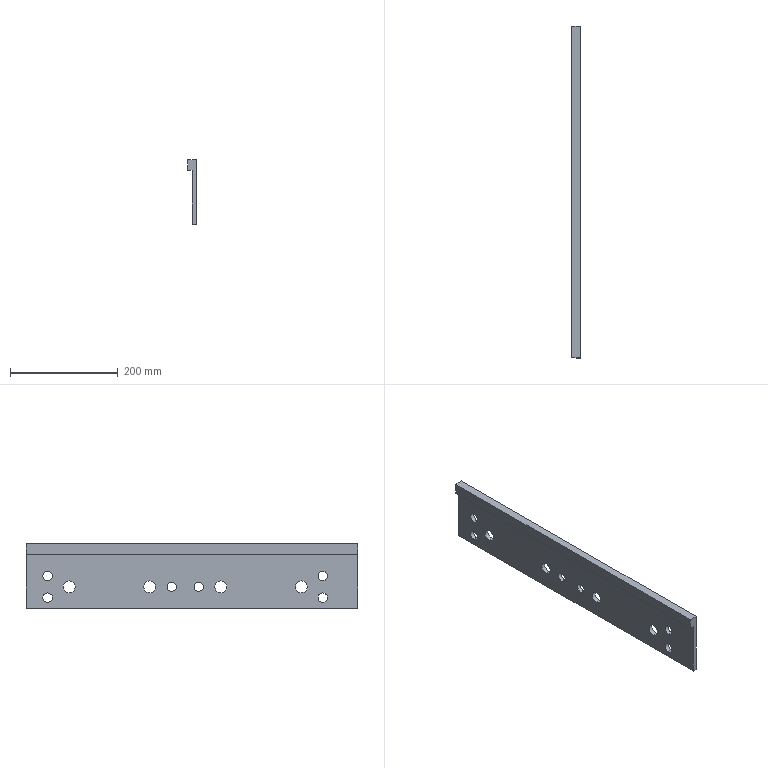Component | SolidWorks | JF21-80.1-1-3(_)-1-SOLID67-1 | 1 solid | 28 faces | box 15 x 615 x 120 mm | volume 623522 mm3 | cylinder 20 | plane 8 | commonest cylinder face diameters 17.5 x12 22 x8
STEP:
#1=COLOUR_RGB('',0.7922,0.8196,0.9333);
#2=FILL_AREA_STYLE_COLOUR('',#1);
#3=FILL_AREA_STYLE('',(#2));
#4=SURFACE_STYLE_FILL_AREA(#3);
#5=SURFACE_SIDE_STYLE('',(#4));
#6=SURFACE_STYLE_USAGE(.BOTH.,#5);
#7=PRESENTATION_STYLE_ASSIGNMENT((#6));
#8=CARTESIAN_POINT('',(15.453,-16.339,5.236));
#9=VERTEX_POINT('',#8);
#10=CARTESIAN_POINT('',(15.453,-16.339,4.37));
#11=VERTEX_POINT('',#10);
#12=CARTESIAN_POINT('',(15.453,-16.339,4.803));
#13=DIRECTION('',(1.,0.,0.));
#14=DIRECTION('',(0.,0.,-1.));
#15=AXIS2_PLACEMENT_3D('',#12,#13,#14);
#16=CIRCLE('',#15,0.4331);
#17=EDGE_CURVE('',#9,#11,#16,.T.);
#18=ORIENTED_EDGE('',*,*,#17,.F.);
#19=CARTESIAN_POINT('',(15.748,-16.339,5.236));
#20=VERTEX_POINT('',#19);
#21=CARTESIAN_POINT('',(17.323,-16.339,5.236));
#22=DIRECTION('',(-1.,0.,0.));
#23=VECTOR('',#22,39.37);
#24=LINE('',#21,#23);
#25=EDGE_CURVE('',#20,#9,#24,.T.);
#26=ORIENTED_EDGE('',*,*,#25,.F.);
#27=CARTESIAN_POINT('',(15.748,-16.339,4.37));
#28=VERTEX_POINT('',#27);
#29=CARTESIAN_POINT('',(15.748,-16.339,4.803));
#30=DIRECTION('',(1.,0.,0.));
#31=DIRECTION('',(0.,0.,-1.));
#32=AXIS2_PLACEMENT_3D('',#29,#30,#31);
#33=CIRCLE('',#32,0.4331);
#34=EDGE_CURVE('',#20,#28,#33,.T.);
#35=ORIENTED_EDGE('',*,*,#34,.T.);
#36=CARTESIAN_POINT('',(17.323,-16.339,4.37));
#37=DIRECTION('',(-1.,0.,0.));
#38=VECTOR('',#37,39.37);
#39=LINE('',#36,#38);
#40=EDGE_CURVE('',#28,#11,#39,.T.);
#41=ORIENTED_EDGE('',*,*,#40,.T.);
#42=EDGE_LOOP('',(#18,#26,#35,#41));
#43=FACE_OUTER_BOUND('',#42,.T.);
#44=CARTESIAN_POINT('',(17.323,-16.339,4.803));
#45=DIRECTION('',(1.,0.,0.));
#46=DIRECTION('',(0.,0.,1.));
#47=AXIS2_PLACEMENT_3D('',#44,#45,#46);
#48=CYLINDRICAL_SURFACE('',#47,0.4331);
#49=ADVANCED_FACE('',(#43),#48,.F.);
#50=CARTESIAN_POINT('',(15.453,-22.205,5.236));
#51=VERTEX_POINT('',#50);
#52=CARTESIAN_POINT('',(15.453,-22.205,4.37));
#53=VERTEX_POINT('',#52);
#54=CARTESIAN_POINT('',(15.453,-22.205,4.803));
#55=DIRECTION('',(1.,0.,0.));
#56=DIRECTION('',(0.,0.,-1.));
#57=AXIS2_PLACEMENT_3D('',#54,#55,#56);
#58=CIRCLE('',#57,0.4331);
#59=EDGE_CURVE('',#51,#53,#58,.T.);
#60=ORIENTED_EDGE('',*,*,#59,.F.);
#61=CARTESIAN_POINT('',(15.748,-22.205,5.236));
#62=VERTEX_POINT('',#61);
#63=CARTESIAN_POINT('',(17.323,-22.205,5.236));
#64=DIRECTION('',(-1.,0.,0.));
#65=VECTOR('',#64,39.37);
#66=LINE('',#63,#65);
#67=EDGE_CURVE('',#62,#51,#66,.T.);
#68=ORIENTED_EDGE('',*,*,#67,.F.);
#69=CARTESIAN_POINT('',(15.748,-22.205,4.37));
#70=VERTEX_POINT('',#69);
#71=CARTESIAN_POINT('',(15.748,-22.205,4.803));
#72=DIRECTION('',(1.,0.,0.));
#73=DIRECTION('',(0.,0.,-1.));
#74=AXIS2_PLACEMENT_3D('',#71,#72,#73);
#75=CIRCLE('',#74,0.4331);
#76=EDGE_CURVE('',#62,#70,#75,.T.);
#77=ORIENTED_EDGE('',*,*,#76,.T.);
#78=CARTESIAN_POINT('',(17.323,-22.205,4.37));
#79=DIRECTION('',(-1.,0.,0.));
#80=VECTOR('',#79,39.37);
#81=LINE('',#78,#80);
#82=EDGE_CURVE('',#70,#53,#81,.T.);
#83=ORIENTED_EDGE('',*,*,#82,.T.);
#84=EDGE_LOOP('',(#60,#68,#77,#83));
#85=FACE_OUTER_BOUND('',#84,.T.);
#86=CARTESIAN_POINT('',(17.323,-22.205,4.803));
#87=DIRECTION('',(1.,0.,0.));
#88=DIRECTION('',(0.,0.,1.));
#89=AXIS2_PLACEMENT_3D('',#86,#87,#88);
#90=CYLINDRICAL_SURFACE('',#89,0.4331);
#91=ADVANCED_FACE('',(#85),#90,.F.);
#92=CARTESIAN_POINT('',(15.453,-27.402,5.236));
#93=VERTEX_POINT('',#92);
#94=CARTESIAN_POINT('',(15.453,-27.402,4.37));
#95=VERTEX_POINT('',#94);
#96=CARTESIAN_POINT('',(15.453,-27.402,4.803));
#97=DIRECTION('',(1.,0.,0.));
#98=DIRECTION('',(0.,0.,-1.));
#99=AXIS2_PLACEMENT_3D('',#96,#97,#98);
#100=CIRCLE('',#99,0.4331);
#101=EDGE_CURVE('',#93,#95,#100,.T.);
#102=ORIENTED_EDGE('',*,*,#101,.F.);
#103=CARTESIAN_POINT('',(15.748,-27.402,5.236));
#104=VERTEX_POINT('',#103);
#105=CARTESIAN_POINT('',(17.323,-27.402,5.236));
#106=DIRECTION('',(-1.,0.,0.));
#107=VECTOR('',#106,39.37);
#108=LINE('',#105,#107);
#109=EDGE_CURVE('',#104,#93,#108,.T.);
#110=ORIENTED_EDGE('',*,*,#109,.F.);
#111=CARTESIAN_POINT('',(15.748,-27.402,4.37));
#112=VERTEX_POINT('',#111);
#113=CARTESIAN_POINT('',(15.748,-27.402,4.803));
#114=DIRECTION('',(1.,0.,0.));
#115=DIRECTION('',(0.,0.,-1.));
#116=AXIS2_PLACEMENT_3D('',#113,#114,#115);
#117=CIRCLE('',#116,0.4331);
#118=EDGE_CURVE('',#104,#112,#117,.T.);
#119=ORIENTED_EDGE('',*,*,#118,.T.);
#120=CARTESIAN_POINT('',(17.323,-27.402,4.37));
#121=DIRECTION('',(-1.,0.,0.));
#122=VECTOR('',#121,39.37);
#123=LINE('',#120,#122);
#124=EDGE_CURVE('',#112,#95,#123,.T.);
#125=ORIENTED_EDGE('',*,*,#124,.T.);
#126=EDGE_LOOP('',(#102,#110,#119,#125));
#127=FACE_OUTER_BOUND('',#126,.T.);
#128=CARTESIAN_POINT('',(17.323,-27.402,4.803));
#129=DIRECTION('',(1.,0.,0.));
#130=DIRECTION('',(0.,0.,1.));
#131=AXIS2_PLACEMENT_3D('',#128,#129,#130);
#132=CYLINDRICAL_SURFACE('',#131,0.4331);
#133=ADVANCED_FACE('',(#127),#132,.F.);
#134=CARTESIAN_POINT('',(15.453,-33.268,5.236));
#135=VERTEX_POINT('',#134);
#136=CARTESIAN_POINT('',(15.453,-33.268,4.37));
#137=VERTEX_POINT('',#136);
#138=CARTESIAN_POINT('',(15.453,-33.268,4.803));
#139=DIRECTION('',(1.,0.,0.));
#140=DIRECTION('',(0.,0.,-1.));
#141=AXIS2_PLACEMENT_3D('',#138,#139,#140);
#142=CIRCLE('',#141,0.4331);
#143=EDGE_CURVE('',#135,#137,#142,.T.);
#144=ORIENTED_EDGE('',*,*,#143,.F.);
#145=CARTESIAN_POINT('',(15.748,-33.268,5.236));
#146=VERTEX_POINT('',#145);
#147=CARTESIAN_POINT('',(17.323,-33.268,5.236));
#148=DIRECTION('',(-1.,0.,0.));
#149=VECTOR('',#148,39.37);
#150=LINE('',#147,#149);
#151=EDGE_CURVE('',#146,#135,#150,.T.);
#152=ORIENTED_EDGE('',*,*,#151,.F.);
#153=CARTESIAN_POINT('',(15.748,-33.268,4.37));
#154=VERTEX_POINT('',#153);
#155=CARTESIAN_POINT('',(15.748,-33.268,4.803));
#156=DIRECTION('',(1.,0.,0.));
#157=DIRECTION('',(0.,0.,-1.));
#158=AXIS2_PLACEMENT_3D('',#155,#156,#157);
#159=CIRCLE('',#158,0.4331);
#160=EDGE_CURVE('',#146,#154,#159,.T.);
#161=ORIENTED_EDGE('',*,*,#160,.T.);
#162=CARTESIAN_POINT('',(17.323,-33.268,4.37));
#163=DIRECTION('',(-1.,0.,0.));
#164=VECTOR('',#163,39.37);
#165=LINE('',#162,#164);
#166=EDGE_CURVE('',#154,#137,#165,.T.);
#167=ORIENTED_EDGE('',*,*,#166,.T.);
#168=EDGE_LOOP('',(#144,#152,#161,#167));
#169=FACE_OUTER_BOUND('',#168,.T.);
#170=CARTESIAN_POINT('',(17.323,-33.268,4.803));
#171=DIRECTION('',(1.,0.,0.));
#172=DIRECTION('',(0.,0.,1.));
#173=AXIS2_PLACEMENT_3D('',#170,#171,#172);
#174=CYLINDRICAL_SURFACE('',#173,0.4331);
#175=ADVANCED_FACE('',(#169),#174,.F.);
#176=CARTESIAN_POINT('',(15.453,-14.764,5.246));
#177=VERTEX_POINT('',#176);
#178=CARTESIAN_POINT('',(15.453,-14.764,5.935));
#179=VERTEX_POINT('',#178);
#180=CARTESIAN_POINT('',(15.453,-14.764,5.591));
#181=DIRECTION('',(-1.,0.,0.));
#182=DIRECTION('',(0.,0.,1.));
#183=AXIS2_PLACEMENT_3D('',#180,#181,#182);
#184=CIRCLE('',#183,0.3445);
#185=EDGE_CURVE('',#177,#179,#184,.T.);
#186=ORIENTED_EDGE('',*,*,#185,.T.);
#187=CARTESIAN_POINT('',(15.748,-14.764,5.935));
#188=VERTEX_POINT('',#187);
#189=CARTESIAN_POINT('',(17.323,-14.764,5.935));
#190=DIRECTION('',(-1.,0.,0.));
#191=VECTOR('',#190,39.37);
#192=LINE('',#189,#191);
#193=EDGE_CURVE('',#188,#179,#192,.T.);
#194=ORIENTED_EDGE('',*,*,#193,.F.);
#195=CARTESIAN_POINT('',(15.748,-14.764,5.246));
#196=VERTEX_POINT('',#195);
#197=CARTESIAN_POINT('',(15.748,-14.764,5.591));
#198=DIRECTION('',(1.,0.,0.));
#199=DIRECTION('',(0.,0.,-1.));
#200=AXIS2_PLACEMENT_3D('',#197,#198,#199);
#201=CIRCLE('',#200,0.3445);
#202=EDGE_CURVE('',#188,#196,#201,.T.);
#203=ORIENTED_EDGE('',*,*,#202,.T.);
#204=CARTESIAN_POINT('',(17.323,-14.764,5.246));
#205=DIRECTION('',(-1.,0.,0.));
#206=VECTOR('',#205,39.37);
#207=LINE('',#204,#206);
#208=EDGE_CURVE('',#196,#177,#207,.T.);
#209=ORIENTED_EDGE('',*,*,#208,.T.);
#210=EDGE_LOOP('',(#186,#194,#203,#209));
#211=FACE_OUTER_BOUND('',#210,.T.);
#212=CARTESIAN_POINT('',(17.323,-14.764,5.591));
#213=DIRECTION('',(1.,0.,0.));
#214=DIRECTION('',(0.,0.,1.));
#215=AXIS2_PLACEMENT_3D('',#212,#213,#214);
#216=CYLINDRICAL_SURFACE('',#215,0.3445);
#217=ADVANCED_FACE('',(#211),#216,.F.);
#218=CARTESIAN_POINT('',(15.453,-14.764,3.671));
#219=VERTEX_POINT('',#218);
#220=CARTESIAN_POINT('',(15.453,-14.764,4.36));
#221=VERTEX_POINT('',#220);
#222=CARTESIAN_POINT('',(15.453,-14.764,4.016));
#223=DIRECTION('',(-1.,0.,0.));
#224=DIRECTION('',(0.,0.,1.));
#225=AXIS2_PLACEMENT_3D('',#222,#223,#224);
#226=CIRCLE('',#225,0.3445);
#227=EDGE_CURVE('',#219,#221,#226,.T.);
#228=ORIENTED_EDGE('',*,*,#227,.T.);
#229=CARTESIAN_POINT('',(15.748,-14.764,4.36));
#230=VERTEX_POINT('',#229);
#231=CARTESIAN_POINT('',(17.323,-14.764,4.36));
#232=DIRECTION('',(-1.,0.,0.));
#233=VECTOR('',#232,39.37);
#234=LINE('',#231,#233);
#235=EDGE_CURVE('',#230,#221,#234,.T.);
#236=ORIENTED_EDGE('',*,*,#235,.F.);
#237=CARTESIAN_POINT('',(15.748,-14.764,3.671));
#238=VERTEX_POINT('',#237);
#239=CARTESIAN_POINT('',(15.748,-14.764,4.016));
#240=DIRECTION('',(1.,0.,0.));
#241=DIRECTION('',(0.,0.,-1.));
#242=AXIS2_PLACEMENT_3D('',#239,#240,#241);
#243=CIRCLE('',#242,0.3445);
#244=EDGE_CURVE('',#230,#238,#243,.T.);
#245=ORIENTED_EDGE('',*,*,#244,.T.);
#246=CARTESIAN_POINT('',(17.323,-14.764,3.671));
#247=DIRECTION('',(-1.,0.,0.));
#248=VECTOR('',#247,39.37);
#249=LINE('',#246,#248);
#250=EDGE_CURVE('',#238,#219,#249,.T.);
#251=ORIENTED_EDGE('',*,*,#250,.T.);
#252=EDGE_LOOP('',(#228,#236,#245,#251));
#253=FACE_OUTER_BOUND('',#252,.T.);
#254=CARTESIAN_POINT('',(17.323,-14.764,4.016));
#255=DIRECTION('',(1.,0.,0.));
#256=DIRECTION('',(0.,0.,1.));
#257=AXIS2_PLACEMENT_3D('',#254,#255,#256);
#258=CYLINDRICAL_SURFACE('',#257,0.3445);
#259=ADVANCED_FACE('',(#253),#258,.F.);
#260=CARTESIAN_POINT('',(15.453,-23.819,4.459));
#261=VERTEX_POINT('',#260);
#262=CARTESIAN_POINT('',(15.453,-23.819,5.148));
#263=VERTEX_POINT('',#262);
#264=CARTESIAN_POINT('',(15.453,-23.819,4.803));
#265=DIRECTION('',(-1.,0.,0.));
#266=DIRECTION('',(0.,0.,1.));
#267=AXIS2_PLACEMENT_3D('',#264,#265,#266);
#268=CIRCLE('',#267,0.3445);
#269=EDGE_CURVE('',#261,#263,#268,.T.);
#270=ORIENTED_EDGE('',*,*,#269,.T.);
#271=CARTESIAN_POINT('',(15.748,-23.819,5.148));
#272=VERTEX_POINT('',#271);
#273=CARTESIAN_POINT('',(17.323,-23.819,5.148));
#274=DIRECTION('',(-1.,0.,0.));
#275=VECTOR('',#274,39.37);
#276=LINE('',#273,#275);
#277=EDGE_CURVE('',#272,#263,#276,.T.);
#278=ORIENTED_EDGE('',*,*,#277,.F.);
#279=CARTESIAN_POINT('',(15.748,-23.819,4.459));
#280=VERTEX_POINT('',#279);
#281=CARTESIAN_POINT('',(15.748,-23.819,4.803));
#282=DIRECTION('',(1.,0.,0.));
#283=DIRECTION('',(0.,0.,-1.));
#284=AXIS2_PLACEMENT_3D('',#281,#282,#283);
#285=CIRCLE('',#284,0.3445);
#286=EDGE_CURVE('',#272,#280,#285,.T.);
#287=ORIENTED_EDGE('',*,*,#286,.T.);
#288=CARTESIAN_POINT('',(17.323,-23.819,4.459));
#289=DIRECTION('',(-1.,0.,0.));
#290=VECTOR('',#289,39.37);
#291=LINE('',#288,#290);
#292=EDGE_CURVE('',#280,#261,#291,.T.);
#293=ORIENTED_EDGE('',*,*,#292,.T.);
#294=EDGE_LOOP('',(#270,#278,#287,#293));
#295=FACE_OUTER_BOUND('',#294,.T.);
#296=CARTESIAN_POINT('',(17.323,-23.819,4.803));
#297=DIRECTION('',(1.,0.,0.));
#298=DIRECTION('',(0.,0.,1.));
#299=AXIS2_PLACEMENT_3D('',#296,#297,#298);
#300=CYLINDRICAL_SURFACE('',#299,0.3445);
#301=ADVANCED_FACE('',(#295),#300,.F.);
#302=CARTESIAN_POINT('',(15.453,-25.787,4.459));
#303=VERTEX_POINT('',#302);
#304=CARTESIAN_POINT('',(15.453,-25.787,5.148));
#305=VERTEX_POINT('',#304);
#306=CARTESIAN_POINT('',(15.453,-25.787,4.803));
#307=DIRECTION('',(-1.,0.,0.));
#308=DIRECTION('',(0.,0.,1.));
#309=AXIS2_PLACEMENT_3D('',#306,#307,#308);
#310=CIRCLE('',#309,0.3445);
#311=EDGE_CURVE('',#303,#305,#310,.T.);
#312=ORIENTED_EDGE('',*,*,#311,.T.);
#313=CARTESIAN_POINT('',(15.748,-25.787,5.148));
#314=VERTEX_POINT('',#313);
#315=CARTESIAN_POINT('',(17.323,-25.787,5.148));
#316=DIRECTION('',(-1.,0.,0.));
#317=VECTOR('',#316,39.37);
#318=LINE('',#315,#317);
#319=EDGE_CURVE('',#314,#305,#318,.T.);
#320=ORIENTED_EDGE('',*,*,#319,.F.);
#321=CARTESIAN_POINT('',(15.748,-25.787,4.459));
#322=VERTEX_POINT('',#321);
#323=CARTESIAN_POINT('',(15.748,-25.787,4.803));
#324=DIRECTION('',(1.,0.,0.));
#325=DIRECTION('',(0.,0.,-1.));
#326=AXIS2_PLACEMENT_3D('',#323,#324,#325);
#327=CIRCLE('',#326,0.3445);
#328=EDGE_CURVE('',#314,#322,#327,.T.);
#329=ORIENTED_EDGE('',*,*,#328,.T.);
#330=CARTESIAN_POINT('',(17.323,-25.787,4.459));
#331=DIRECTION('',(-1.,0.,0.));
#332=VECTOR('',#331,39.37);
#333=LINE('',#330,#332);
#334=EDGE_CURVE('',#322,#303,#333,.T.);
#335=ORIENTED_EDGE('',*,*,#334,.T.);
#336=EDGE_LOOP('',(#312,#320,#329,#335));
#337=FACE_OUTER_BOUND('',#336,.T.);
#338=CARTESIAN_POINT('',(17.323,-25.787,4.803));
#339=DIRECTION('',(1.,0.,0.));
#340=DIRECTION('',(0.,0.,1.));
#341=AXIS2_PLACEMENT_3D('',#338,#339,#340);
#342=CYLINDRICAL_SURFACE('',#341,0.3445);
#343=ADVANCED_FACE('',(#337),#342,.F.);
#344=CARTESIAN_POINT('',(15.453,-34.843,5.246));
#345=VERTEX_POINT('',#344);
#346=CARTESIAN_POINT('',(15.453,-34.843,5.935));
#347=VERTEX_POINT('',#346);
#348=CARTESIAN_POINT('',(15.453,-34.843,5.591));
#349=DIRECTION('',(-1.,0.,0.));
#350=DIRECTION('',(0.,0.,1.));
#351=AXIS2_PLACEMENT_3D('',#348,#349,#350);
#352=CIRCLE('',#351,0.3445);
#353=EDGE_CURVE('',#345,#347,#352,.T.);
#354=ORIENTED_EDGE('',*,*,#353,.T.);
#355=CARTESIAN_POINT('',(15.748,-34.843,5.935));
#356=VERTEX_POINT('',#355);
#357=CARTESIAN_POINT('',(17.323,-34.843,5.935));
#358=DIRECTION('',(-1.,0.,0.));
#359=VECTOR('',#358,39.37);
#360=LINE('',#357,#359);
#361=EDGE_CURVE('',#356,#347,#360,.T.);
#362=ORIENTED_EDGE('',*,*,#361,.F.);
#363=CARTESIAN_POINT('',(15.748,-34.843,5.246));
#364=VERTEX_POINT('',#363);
#365=CARTESIAN_POINT('',(15.748,-34.843,5.591));
#366=DIRECTION('',(1.,0.,0.));
#367=DIRECTION('',(0.,0.,-1.));
#368=AXIS2_PLACEMENT_3D('',#365,#366,#367);
#369=CIRCLE('',#368,0.3445);
#370=EDGE_CURVE('',#356,#364,#369,.T.);
#371=ORIENTED_EDGE('',*,*,#370,.T.);
#372=CARTESIAN_POINT('',(17.323,-34.843,5.246));
#373=DIRECTION('',(-1.,0.,0.));
#374=VECTOR('',#373,39.37);
#375=LINE('',#372,#374);
#376=EDGE_CURVE('',#364,#345,#375,.T.);
#377=ORIENTED_EDGE('',*,*,#376,.T.);
#378=EDGE_LOOP('',(#354,#362,#371,#377));
#379=FACE_OUTER_BOUND('',#378,.T.);
#380=CARTESIAN_POINT('',(17.323,-34.843,5.591));
#381=DIRECTION('',(1.,0.,0.));
#382=DIRECTION('',(0.,0.,1.));
#383=AXIS2_PLACEMENT_3D('',#380,#381,#382);
#384=CYLINDRICAL_SURFACE('',#383,0.3445);
#385=ADVANCED_FACE('',(#379),#384,.F.);
#386=CARTESIAN_POINT('',(15.453,-34.843,3.671));
#387=VERTEX_POINT('',#386);
#388=CARTESIAN_POINT('',(15.453,-34.843,4.36));
#389=VERTEX_POINT('',#388);
#390=CARTESIAN_POINT('',(15.453,-34.843,4.016));
#391=DIRECTION('',(-1.,0.,0.));
#392=DIRECTION('',(0.,0.,1.));
#393=AXIS2_PLACEMENT_3D('',#390,#391,#392);
#394=CIRCLE('',#393,0.3445);
#395=EDGE_CURVE('',#387,#389,#394,.T.);
#396=ORIENTED_EDGE('',*,*,#395,.T.);
#397=CARTESIAN_POINT('',(15.748,-34.843,4.36));
#398=VERTEX_POINT('',#397);
#399=CARTESIAN_POINT('',(17.323,-34.843,4.36));
#400=DIRECTION('',(-1.,0.,0.));
#401=VECTOR('',#400,39.37);
#402=LINE('',#399,#401);
#403=EDGE_CURVE('',#398,#389,#402,.T.);
#404=ORIENTED_EDGE('',*,*,#403,.F.);
#405=CARTESIAN_POINT('',(15.748,-34.843,3.671));
#406=VERTEX_POINT('',#405);
#407=CARTESIAN_POINT('',(15.748,-34.843,4.016));
#408=DIRECTION('',(1.,0.,0.));
#409=DIRECTION('',(0.,0.,-1.));
#410=AXIS2_PLACEMENT_3D('',#407,#408,#409);
#411=CIRCLE('',#410,0.3445);
#412=EDGE_CURVE('',#398,#406,#411,.T.);
#413=ORIENTED_EDGE('',*,*,#412,.T.);
#414=CARTESIAN_POINT('',(17.323,-34.843,3.671));
#415=DIRECTION('',(-1.,0.,0.));
#416=VECTOR('',#415,39.37);
#417=LINE('',#414,#416);
#418=EDGE_CURVE('',#406,#387,#417,.T.);
#419=ORIENTED_EDGE('',*,*,#418,.T.);
#420=EDGE_LOOP('',(#396,#404,#413,#419));
#421=FACE_OUTER_BOUND('',#420,.T.);
#422=CARTESIAN_POINT('',(17.323,-34.843,4.016));
#423=DIRECTION('',(1.,0.,0.));
#424=DIRECTION('',(0.,0.,1.));
#425=AXIS2_PLACEMENT_3D('',#422,#423,#424);
#426=CYLINDRICAL_SURFACE('',#425,0.3445);
#427=ADVANCED_FACE('',(#421),#426,.F.);
#428=CARTESIAN_POINT('',(15.748,-16.339,4.803));
#429=DIRECTION('',(1.,0.,0.));
#430=DIRECTION('',(0.,0.,-1.));
#431=AXIS2_PLACEMENT_3D('',#428,#429,#430);
#432=CIRCLE('',#431,0.4331);
#433=EDGE_CURVE('',#28,#20,#432,.T.);
#434=ORIENTED_EDGE('',*,*,#433,.F.);
#435=ORIENTED_EDGE('',*,*,#34,.F.);
#436=EDGE_LOOP('',(#434,#435));
#437=FACE_BOUND('',#436,.T.);
#438=CARTESIAN_POINT('',(15.748,-22.205,4.803));
#439=DIRECTION('',(1.,0.,0.));
#440=DIRECTION('',(0.,0.,-1.));
#441=AXIS2_PLACEMENT_3D('',#438,#439,#440);
#442=CIRCLE('',#441,0.4331);
#443=EDGE_CURVE('',#70,#62,#442,.T.);
#444=ORIENTED_EDGE('',*,*,#443,.F.);
#445=ORIENTED_EDGE('',*,*,#76,.F.);
#446=EDGE_LOOP('',(#444,#445));
#447=FACE_BOUND('',#446,.T.);
#448=CARTESIAN_POINT('',(15.748,-27.402,4.803));
#449=DIRECTION('',(1.,0.,0.));
#450=DIRECTION('',(0.,0.,-1.));
#451=AXIS2_PLACEMENT_3D('',#448,#449,#450);
#452=CIRCLE('',#451,0.4331);
#453=EDGE_CURVE('',#112,#104,#452,.T.);
#454=ORIENTED_EDGE('',*,*,#453,.F.);
#455=ORIENTED_EDGE('',*,*,#118,.F.);
#456=EDGE_LOOP('',(#454,#455));
#457=FACE_BOUND('',#456,.T.);
#458=CARTESIAN_POINT('',(15.748,-33.268,4.803));
#459=DIRECTION('',(1.,0.,0.));
#460=DIRECTION('',(0.,0.,-1.));
#461=AXIS2_PLACEMENT_3D('',#458,#459,#460);
#462=CIRCLE('',#461,0.4331);
#463=EDGE_CURVE('',#154,#146,#462,.T.);
#464=ORIENTED_EDGE('',*,*,#463,.F.);
#465=ORIENTED_EDGE('',*,*,#160,.F.);
#466=EDGE_LOOP('',(#464,#465));
#467=FACE_BOUND('',#466,.T.);
#468=CARTESIAN_POINT('',(15.748,-14.764,5.591));
#469=DIRECTION('',(1.,0.,0.));
#470=DIRECTION('',(0.,0.,-1.));
#471=AXIS2_PLACEMENT_3D('',#468,#469,#470);
#472=CIRCLE('',#471,0.3445);
#473=EDGE_CURVE('',#196,#188,#472,.T.);
#474=ORIENTED_EDGE('',*,*,#473,.F.);
#475=ORIENTED_EDGE('',*,*,#202,.F.);
#476=EDGE_LOOP('',(#474,#475));
#477=FACE_BOUND('',#476,.T.);
#478=CARTESIAN_POINT('',(15.748,-14.764,4.016));
#479=DIRECTION('',(1.,0.,0.));
#480=DIRECTION('',(0.,0.,-1.));
#481=AXIS2_PLACEMENT_3D('',#478,#479,#480);
#482=CIRCLE('',#481,0.3445);
#483=EDGE_CURVE('',#238,#230,#482,.T.);
#484=ORIENTED_EDGE('',*,*,#483,.F.);
#485=ORIENTED_EDGE('',*,*,#244,.F.);
#486=EDGE_LOOP('',(#484,#485));
#487=FACE_BOUND('',#486,.T.);
#488=CARTESIAN_POINT('',(15.748,-23.819,4.803));
#489=DIRECTION('',(1.,0.,0.));
#490=DIRECTION('',(0.,0.,-1.));
#491=AXIS2_PLACEMENT_3D('',#488,#489,#490);
#492=CIRCLE('',#491,0.3445);
#493=EDGE_CURVE('',#280,#272,#492,.T.);
#494=ORIENTED_EDGE('',*,*,#493,.F.);
#495=ORIENTED_EDGE('',*,*,#286,.F.);
#496=EDGE_LOOP('',(#494,#495));
#497=FACE_BOUND('',#496,.T.);
#498=CARTESIAN_POINT('',(15.748,-25.787,4.803));
#499=DIRECTION('',(1.,0.,0.));
#500=DIRECTION('',(0.,0.,-1.));
#501=AXIS2_PLACEMENT_3D('',#498,#499,#500);
#502=CIRCLE('',#501,0.3445);
#503=EDGE_CURVE('',#322,#314,#502,.T.);
#504=ORIENTED_EDGE('',*,*,#503,.F.);
#505=ORIENTED_EDGE('',*,*,#328,.F.);
#506=EDGE_LOOP('',(#504,#505));
#507=FACE_BOUND('',#506,.T.);
#508=CARTESIAN_POINT('',(15.748,-34.843,5.591));
#509=DIRECTION('',(1.,0.,0.));
#510=DIRECTION('',(0.,0.,-1.));
#511=AXIS2_PLACEMENT_3D('',#508,#509,#510);
#512=CIRCLE('',#511,0.3445);
#513=EDGE_CURVE('',#364,#356,#512,.T.);
#514=ORIENTED_EDGE('',*,*,#513,.F.);
#515=ORIENTED_EDGE('',*,*,#370,.F.);
#516=EDGE_LOOP('',(#514,#515));
#517=FACE_BOUND('',#516,.T.);
#518=CARTESIAN_POINT('',(15.748,-34.843,4.016));
#519=DIRECTION('',(1.,0.,0.));
#520=DIRECTION('',(0.,0.,-1.));
#521=AXIS2_PLACEMENT_3D('',#518,#519,#520);
#522=CIRCLE('',#521,0.3445);
#523=EDGE_CURVE('',#406,#398,#522,.T.);
#524=ORIENTED_EDGE('',*,*,#523,.F.);
#525=ORIENTED_EDGE('',*,*,#412,.F.);
#526=EDGE_LOOP('',(#524,#525));
#527=FACE_BOUND('',#526,.T.);
#528=CARTESIAN_POINT('',(15.748,-37.402,3.228));
#529=VERTEX_POINT('',#528);
#530=CARTESIAN_POINT('',(15.748,-37.402,7.953));
#531=VERTEX_POINT('',#530);
#532=CARTESIAN_POINT('',(15.748,-37.402,7.953));
#533=DIRECTION('',(0.,-0.,1.));
#534=VECTOR('',#533,39.37);
#535=LINE('',#532,#534);
#536=EDGE_CURVE('',#529,#531,#535,.T.);
#537=ORIENTED_EDGE('',*,*,#536,.F.);
#538=CARTESIAN_POINT('',(15.748,-13.189,3.228));
#539=VERTEX_POINT('',#538);
#540=CARTESIAN_POINT('',(15.748,-13.189,3.228));
#541=DIRECTION('',(0.,-1.,-0.));
#542=VECTOR('',#541,39.37);
#543=LINE('',#540,#542);
#544=EDGE_CURVE('',#539,#529,#543,.T.);
#545=ORIENTED_EDGE('',*,*,#544,.F.);
#546=CARTESIAN_POINT('',(15.748,-13.189,7.953));
#547=VERTEX_POINT('',#546);
#548=CARTESIAN_POINT('',(15.748,-13.189,7.953));
#549=DIRECTION('',(0.,-0.,1.));
#550=VECTOR('',#549,39.37);
#551=LINE('',#548,#550);
#552=EDGE_CURVE('',#539,#547,#551,.T.);
#553=ORIENTED_EDGE('',*,*,#552,.T.);
#554=CARTESIAN_POINT('',(15.748,-13.189,7.953));
#555=DIRECTION('',(0.,-1.,-0.));
#556=VECTOR('',#555,39.37);
#557=LINE('',#554,#556);
#558=EDGE_CURVE('',#547,#531,#557,.T.);
#559=ORIENTED_EDGE('',*,*,#558,.T.);
#560=EDGE_LOOP('',(#537,#545,#553,#559));
#561=FACE_OUTER_BOUND('',#560,.T.);
#562=CARTESIAN_POINT('',(15.748,-13.189,7.953));
#563=DIRECTION('',(1.,0.,0.));
#564=DIRECTION('',(0.,0.,1.));
#565=AXIS2_PLACEMENT_3D('',#562,#563,#564);
#566=PLANE('',#565);
#567=ADVANCED_FACE('',(#437,#447,#457,#467,#477,#487,#497,#507,#517,#527,#561),#566,.T.);
#568=CARTESIAN_POINT('',(15.453,-37.402,3.228));
#569=VERTEX_POINT('',#568);
#570=CARTESIAN_POINT('',(15.748,-37.402,3.228));
#571=DIRECTION('',(1.,0.,0.));
#572=VECTOR('',#571,39.37);
#573=LINE('',#570,#572);
#574=EDGE_CURVE('',#569,#529,#573,.T.);
#575=ORIENTED_EDGE('',*,*,#574,.F.);
#576=CARTESIAN_POINT('',(15.453,-13.189,3.228));
#577=VERTEX_POINT('',#576);
#578=CARTESIAN_POINT('',(15.453,-13.189,3.228));
#579=DIRECTION('',(0.,-1.,-0.));
#580=VECTOR('',#579,39.37);
#581=LINE('',#578,#580);
#582=EDGE_CURVE('',#577,#569,#581,.T.);
#583=ORIENTED_EDGE('',*,*,#582,.F.);
#584=CARTESIAN_POINT('',(15.748,-13.189,3.228));
#585=DIRECTION('',(1.,0.,0.));
#586=VECTOR('',#585,39.37);
#587=LINE('',#584,#586);
#588=EDGE_CURVE('',#577,#539,#587,.T.);
#589=ORIENTED_EDGE('',*,*,#588,.T.);
#590=ORIENTED_EDGE('',*,*,#544,.T.);
#591=EDGE_LOOP('',(#575,#583,#589,#590));
#592=FACE_OUTER_BOUND('',#591,.T.);
#593=CARTESIAN_POINT('',(15.748,-13.189,3.228));
#594=DIRECTION('',(0.,0.,-1.));
#595=DIRECTION('',(0.,-1.,-0.));
#596=AXIS2_PLACEMENT_3D('',#593,#594,#595);
#597=PLANE('',#596);
#598=ADVANCED_FACE('',(#592),#597,.T.);
#599=CARTESIAN_POINT('',(15.453,-16.339,4.803));
#600=DIRECTION('',(1.,0.,0.));
#601=DIRECTION('',(0.,0.,-1.));
#602=AXIS2_PLACEMENT_3D('',#599,#600,#601);
#603=CIRCLE('',#602,0.4331);
#604=EDGE_CURVE('',#11,#9,#603,.T.);
#605=ORIENTED_EDGE('',*,*,#604,.T.);
#606=ORIENTED_EDGE('',*,*,#17,.T.);
#607=EDGE_LOOP('',(#605,#606));
#608=FACE_BOUND('',#607,.T.);
#609=CARTESIAN_POINT('',(15.453,-22.205,4.803));
#610=DIRECTION('',(1.,0.,0.));
#611=DIRECTION('',(0.,0.,-1.));
#612=AXIS2_PLACEMENT_3D('',#609,#610,#611);
#613=CIRCLE('',#612,0.4331);
#614=EDGE_CURVE('',#53,#51,#613,.T.);
#615=ORIENTED_EDGE('',*,*,#614,.T.);
#616=ORIENTED_EDGE('',*,*,#59,.T.);
#617=EDGE_LOOP('',(#615,#616));
#618=FACE_BOUND('',#617,.T.);
#619=CARTESIAN_POINT('',(15.453,-27.402,4.803));
#620=DIRECTION('',(1.,0.,0.));
#621=DIRECTION('',(0.,0.,-1.));
#622=AXIS2_PLACEMENT_3D('',#619,#620,#621);
#623=CIRCLE('',#622,0.4331);
#624=EDGE_CURVE('',#95,#93,#623,.T.);
#625=ORIENTED_EDGE('',*,*,#624,.T.);
#626=ORIENTED_EDGE('',*,*,#101,.T.);
#627=EDGE_LOOP('',(#625,#626));
#628=FACE_BOUND('',#627,.T.);
#629=CARTESIAN_POINT('',(15.453,-33.268,4.803));
#630=DIRECTION('',(1.,0.,0.));
#631=DIRECTION('',(0.,0.,-1.));
#632=AXIS2_PLACEMENT_3D('',#629,#630,#631);
#633=CIRCLE('',#632,0.4331);
#634=EDGE_CURVE('',#137,#135,#633,.T.);
#635=ORIENTED_EDGE('',*,*,#634,.T.);
#636=ORIENTED_EDGE('',*,*,#143,.T.);
#637=EDGE_LOOP('',(#635,#636));
#638=FACE_BOUND('',#637,.T.);
#639=ORIENTED_EDGE('',*,*,#185,.F.);
#640=CARTESIAN_POINT('',(15.453,-14.764,5.591));
#641=DIRECTION('',(-1.,0.,0.));
#642=DIRECTION('',(0.,0.,1.));
#643=AXIS2_PLACEMENT_3D('',#640,#641,#642);
#644=CIRCLE('',#643,0.3445);
#645=EDGE_CURVE('',#179,#177,#644,.T.);
#646=ORIENTED_EDGE('',*,*,#645,.F.);
#647=EDGE_LOOP('',(#639,#646));
#648=FACE_BOUND('',#647,.T.);
#649=ORIENTED_EDGE('',*,*,#227,.F.);
#650=CARTESIAN_POINT('',(15.453,-14.764,4.016));
#651=DIRECTION('',(-1.,0.,0.));
#652=DIRECTION('',(0.,0.,1.));
#653=AXIS2_PLACEMENT_3D('',#650,#651,#652);
#654=CIRCLE('',#653,0.3445);
#655=EDGE_CURVE('',#221,#219,#654,.T.);
#656=ORIENTED_EDGE('',*,*,#655,.F.);
#657=EDGE_LOOP('',(#649,#656));
#658=FACE_BOUND('',#657,.T.);
#659=ORIENTED_EDGE('',*,*,#269,.F.);
#660=CARTESIAN_POINT('',(15.453,-23.819,4.803));
#661=DIRECTION('',(-1.,0.,0.));
#662=DIRECTION('',(0.,0.,1.));
#663=AXIS2_PLACEMENT_3D('',#660,#661,#662);
#664=CIRCLE('',#663,0.3445);
#665=EDGE_CURVE('',#263,#261,#664,.T.);
#666=ORIENTED_EDGE('',*,*,#665,.F.);
#667=EDGE_LOOP('',(#659,#666));
#668=FACE_BOUND('',#667,.T.);
#669=ORIENTED_EDGE('',*,*,#311,.F.);
#670=CARTESIAN_POINT('',(15.453,-25.787,4.803));
#671=DIRECTION('',(-1.,0.,0.));
#672=DIRECTION('',(0.,0.,1.));
#673=AXIS2_PLACEMENT_3D('',#670,#671,#672);
#674=CIRCLE('',#673,0.3445);
#675=EDGE_CURVE('',#305,#303,#674,.T.);
#676=ORIENTED_EDGE('',*,*,#675,.F.);
#677=EDGE_LOOP('',(#669,#676));
#678=FACE_BOUND('',#677,.T.);
#679=ORIENTED_EDGE('',*,*,#353,.F.);
#680=CARTESIAN_POINT('',(15.453,-34.843,5.591));
#681=DIRECTION('',(-1.,0.,0.));
#682=DIRECTION('',(0.,0.,1.));
#683=AXIS2_PLACEMENT_3D('',#680,#681,#682);
#684=CIRCLE('',#683,0.3445);
#685=EDGE_CURVE('',#347,#345,#684,.T.);
#686=ORIENTED_EDGE('',*,*,#685,.F.);
#687=EDGE_LOOP('',(#679,#686));
#688=FACE_BOUND('',#687,.T.);
#689=ORIENTED_EDGE('',*,*,#395,.F.);
#690=CARTESIAN_POINT('',(15.453,-34.843,4.016));
#691=DIRECTION('',(-1.,0.,0.));
#692=DIRECTION('',(0.,0.,1.));
#693=AXIS2_PLACEMENT_3D('',#690,#691,#692);
#694=CIRCLE('',#693,0.3445);
#695=EDGE_CURVE('',#389,#387,#694,.T.);
#696=ORIENTED_EDGE('',*,*,#695,.F.);
#697=EDGE_LOOP('',(#689,#696));
#698=FACE_BOUND('',#697,.T.);
#699=CARTESIAN_POINT('',(15.453,-37.402,7.165));
#700=VERTEX_POINT('',#699);
#701=CARTESIAN_POINT('',(15.453,-37.402,3.228));
#702=DIRECTION('',(0.,0.,-1.));
#703=VECTOR('',#702,39.37);
#704=LINE('',#701,#703);
#705=EDGE_CURVE('',#700,#569,#704,.T.);
#706=ORIENTED_EDGE('',*,*,#705,.F.);
#707=CARTESIAN_POINT('',(15.453,-13.189,7.165));
#708=VERTEX_POINT('',#707);
#709=CARTESIAN_POINT('',(15.453,-13.189,7.165));
#710=DIRECTION('',(0.,-1.,-0.));
#711=VECTOR('',#710,39.37);
#712=LINE('',#709,#711);
#713=EDGE_CURVE('',#708,#700,#712,.T.);
#714=ORIENTED_EDGE('',*,*,#713,.F.);
#715=CARTESIAN_POINT('',(15.453,-13.189,3.228));
#716=DIRECTION('',(0.,0.,-1.));
#717=VECTOR('',#716,39.37);
#718=LINE('',#715,#717);
#719=EDGE_CURVE('',#708,#577,#718,.T.);
#720=ORIENTED_EDGE('',*,*,#719,.T.);
#721=ORIENTED_EDGE('',*,*,#582,.T.);
#722=EDGE_LOOP('',(#706,#714,#720,#721));
#723=FACE_OUTER_BOUND('',#722,.T.);
#724=CARTESIAN_POINT('',(15.453,-13.189,3.228));
#725=DIRECTION('',(-1.,0.,0.));
#726=DIRECTION('',(0.,0.,-1.));
#727=AXIS2_PLACEMENT_3D('',#724,#725,#726);
#728=PLANE('',#727);
#729=ADVANCED_FACE('',(#608,#618,#628,#638,#648,#658,#668,#678,#688,#698,#723),#728,.T.);
#730=CARTESIAN_POINT('',(15.157,-37.402,7.165));
#731=VERTEX_POINT('',#730);
#732=CARTESIAN_POINT('',(15.453,-37.402,7.165));
#733=DIRECTION('',(1.,0.,0.));
#734=VECTOR('',#733,39.37);
#735=LINE('',#732,#734);
#736=EDGE_CURVE('',#731,#700,#735,.T.);
#737=ORIENTED_EDGE('',*,*,#736,.F.);
#738=CARTESIAN_POINT('',(15.157,-13.189,7.165));
#739=VERTEX_POINT('',#738);
#740=CARTESIAN_POINT('',(15.157,-13.189,7.165));
#741=DIRECTION('',(0.,-1.,-0.));
#742=VECTOR('',#741,39.37);
#743=LINE('',#740,#742);
#744=EDGE_CURVE('',#739,#731,#743,.T.);
#745=ORIENTED_EDGE('',*,*,#744,.F.);
#746=CARTESIAN_POINT('',(15.453,-13.189,7.165));
#747=DIRECTION('',(1.,0.,0.));
#748=VECTOR('',#747,39.37);
#749=LINE('',#746,#748);
#750=EDGE_CURVE('',#739,#708,#749,.T.);
#751=ORIENTED_EDGE('',*,*,#750,.T.);
#752=ORIENTED_EDGE('',*,*,#713,.T.);
#753=EDGE_LOOP('',(#737,#745,#751,#752));
#754=FACE_OUTER_BOUND('',#753,.T.);
#755=CARTESIAN_POINT('',(15.453,-13.189,7.165));
#756=DIRECTION('',(0.,0.,-1.));
#757=DIRECTION('',(0.,-1.,-0.));
#758=AXIS2_PLACEMENT_3D('',#755,#756,#757);
#759=PLANE('',#758);
#760=ADVANCED_FACE('',(#754),#759,.T.);
#761=CARTESIAN_POINT('',(15.157,-37.402,7.953));
#762=VERTEX_POINT('',#761);
#763=CARTESIAN_POINT('',(15.157,-37.402,7.165));
#764=DIRECTION('',(0.,0.,-1.));
#765=VECTOR('',#764,39.37);
#766=LINE('',#763,#765);
#767=EDGE_CURVE('',#762,#731,#766,.T.);
#768=ORIENTED_EDGE('',*,*,#767,.F.);
#769=CARTESIAN_POINT('',(15.157,-13.189,7.953));
#770=VERTEX_POINT('',#769);
#771=CARTESIAN_POINT('',(15.157,-13.189,7.953));
#772=DIRECTION('',(0.,-1.,-0.));
#773=VECTOR('',#772,39.37);
#774=LINE('',#771,#773);
#775=EDGE_CURVE('',#770,#762,#774,.T.);
#776=ORIENTED_EDGE('',*,*,#775,.F.);
#777=CARTESIAN_POINT('',(15.157,-13.189,7.165));
#778=DIRECTION('',(0.,0.,-1.));
#779=VECTOR('',#778,39.37);
#780=LINE('',#777,#779);
#781=EDGE_CURVE('',#770,#739,#780,.T.);
#782=ORIENTED_EDGE('',*,*,#781,.T.);
#783=ORIENTED_EDGE('',*,*,#744,.T.);
#784=EDGE_LOOP('',(#768,#776,#782,#783));
#785=FACE_OUTER_BOUND('',#784,.T.);
#786=CARTESIAN_POINT('',(15.157,-13.189,7.165));
#787=DIRECTION('',(-1.,0.,0.));
#788=DIRECTION('',(0.,0.,-1.));
#789=AXIS2_PLACEMENT_3D('',#786,#787,#788);
#790=PLANE('',#789);
#791=ADVANCED_FACE('',(#785),#790,.T.);
#792=CARTESIAN_POINT('',(15.157,-37.402,7.953));
#793=DIRECTION('',(-1.,0.,0.));
#794=VECTOR('',#793,39.37);
#795=LINE('',#792,#794);
#796=EDGE_CURVE('',#531,#762,#795,.T.);
#797=ORIENTED_EDGE('',*,*,#796,.F.);
#798=ORIENTED_EDGE('',*,*,#558,.F.);
#799=CARTESIAN_POINT('',(15.157,-13.189,7.953));
#800=DIRECTION('',(-1.,0.,0.));
#801=VECTOR('',#800,39.37);
#802=LINE('',#799,#801);
#803=EDGE_CURVE('',#547,#770,#802,.T.);
#804=ORIENTED_EDGE('',*,*,#803,.T.);
#805=ORIENTED_EDGE('',*,*,#775,.T.);
#806=EDGE_LOOP('',(#797,#798,#804,#805));
#807=FACE_OUTER_BOUND('',#806,.T.);
#808=CARTESIAN_POINT('',(15.157,-13.189,7.953));
#809=DIRECTION('',(0.,-0.,1.));
#810=DIRECTION('',(0.,1.,0.));
#811=AXIS2_PLACEMENT_3D('',#808,#809,#810);
#812=PLANE('',#811);
#813=ADVANCED_FACE('',(#807),#812,.T.);
#814=ORIENTED_EDGE('',*,*,#552,.F.);
#815=ORIENTED_EDGE('',*,*,#588,.F.);
#816=ORIENTED_EDGE('',*,*,#719,.F.);
#817=ORIENTED_EDGE('',*,*,#750,.F.);
#818=ORIENTED_EDGE('',*,*,#781,.F.);
#819=ORIENTED_EDGE('',*,*,#803,.F.);
#820=EDGE_LOOP('',(#814,#815,#816,#817,#818,#819));
#821=FACE_OUTER_BOUND('',#820,.T.);
#822=CARTESIAN_POINT('',(15.748,-13.189,3.228));
#823=DIRECTION('',(0.,1.,0.));
#824=DIRECTION('',(0.,0.,-1.));
#825=AXIS2_PLACEMENT_3D('',#822,#823,#824);
#826=PLANE('',#825);
#827=ADVANCED_FACE('',(#821),#826,.T.);
#828=ORIENTED_EDGE('',*,*,#536,.T.);
#829=ORIENTED_EDGE('',*,*,#796,.T.);
#830=ORIENTED_EDGE('',*,*,#767,.T.);
#831=ORIENTED_EDGE('',*,*,#736,.T.);
#832=ORIENTED_EDGE('',*,*,#705,.T.);
#833=ORIENTED_EDGE('',*,*,#574,.T.);
#834=EDGE_LOOP('',(#828,#829,#830,#831,#832,#833));
#835=FACE_OUTER_BOUND('',#834,.T.);
#836=CARTESIAN_POINT('',(15.748,-37.402,3.228));
#837=DIRECTION('',(0.,1.,0.));
#838=DIRECTION('',(0.,0.,-1.));
#839=AXIS2_PLACEMENT_3D('',#836,#837,#838);
#840=PLANE('',#839);
#841=ADVANCED_FACE('',(#835),#840,.F.);
#842=ORIENTED_EDGE('',*,*,#403,.T.);
#843=ORIENTED_EDGE('',*,*,#695,.T.);
#844=ORIENTED_EDGE('',*,*,#418,.F.);
#845=ORIENTED_EDGE('',*,*,#523,.T.);
#846=EDGE_LOOP('',(#842,#843,#844,#845));
#847=FACE_OUTER_BOUND('',#846,.T.);
#848=CARTESIAN_POINT('',(17.323,-34.843,4.016));
#849=DIRECTION('',(1.,0.,0.));
#850=DIRECTION('',(0.,0.,1.));
#851=AXIS2_PLACEMENT_3D('',#848,#849,#850);
#852=CYLINDRICAL_SURFACE('',#851,0.3445);
#853=ADVANCED_FACE('',(#847),#852,.F.);
#854=ORIENTED_EDGE('',*,*,#361,.T.);
#855=ORIENTED_EDGE('',*,*,#685,.T.);
#856=ORIENTED_EDGE('',*,*,#376,.F.);
#857=ORIENTED_EDGE('',*,*,#513,.T.);
#858=EDGE_LOOP('',(#854,#855,#856,#857));
#859=FACE_OUTER_BOUND('',#858,.T.);
#860=CARTESIAN_POINT('',(17.323,-34.843,5.591));
#861=DIRECTION('',(1.,0.,0.));
#862=DIRECTION('',(0.,0.,1.));
#863=AXIS2_PLACEMENT_3D('',#860,#861,#862);
#864=CYLINDRICAL_SURFACE('',#863,0.3445);
#865=ADVANCED_FACE('',(#859),#864,.F.);
#866=ORIENTED_EDGE('',*,*,#319,.T.);
#867=ORIENTED_EDGE('',*,*,#675,.T.);
#868=ORIENTED_EDGE('',*,*,#334,.F.);
#869=ORIENTED_EDGE('',*,*,#503,.T.);
#870=EDGE_LOOP('',(#866,#867,#868,#869));
#871=FACE_OUTER_BOUND('',#870,.T.);
#872=CARTESIAN_POINT('',(17.323,-25.787,4.803));
#873=DIRECTION('',(1.,0.,0.));
#874=DIRECTION('',(0.,0.,1.));
#875=AXIS2_PLACEMENT_3D('',#872,#873,#874);
#876=CYLINDRICAL_SURFACE('',#875,0.3445);
#877=ADVANCED_FACE('',(#871),#876,.F.);
#878=ORIENTED_EDGE('',*,*,#277,.T.);
#879=ORIENTED_EDGE('',*,*,#665,.T.);
#880=ORIENTED_EDGE('',*,*,#292,.F.);
#881=ORIENTED_EDGE('',*,*,#493,.T.);
#882=EDGE_LOOP('',(#878,#879,#880,#881));
#883=FACE_OUTER_BOUND('',#882,.T.);
#884=CARTESIAN_POINT('',(17.323,-23.819,4.803));
#885=DIRECTION('',(1.,0.,0.));
#886=DIRECTION('',(0.,0.,1.));
#887=AXIS2_PLACEMENT_3D('',#884,#885,#886);
#888=CYLINDRICAL_SURFACE('',#887,0.3445);
#889=ADVANCED_FACE('',(#883),#888,.F.);
#890=ORIENTED_EDGE('',*,*,#235,.T.);
#891=ORIENTED_EDGE('',*,*,#655,.T.);
#892=ORIENTED_EDGE('',*,*,#250,.F.);
#893=ORIENTED_EDGE('',*,*,#483,.T.);
#894=EDGE_LOOP('',(#890,#891,#892,#893));
#895=FACE_OUTER_BOUND('',#894,.T.);
#896=CARTESIAN_POINT('',(17.323,-14.764,4.016));
#897=DIRECTION('',(1.,0.,0.));
#898=DIRECTION('',(0.,0.,1.));
#899=AXIS2_PLACEMENT_3D('',#896,#897,#898);
#900=CYLINDRICAL_SURFACE('',#899,0.3445);
#901=ADVANCED_FACE('',(#895),#900,.F.);
#902=ORIENTED_EDGE('',*,*,#193,.T.);
#903=ORIENTED_EDGE('',*,*,#645,.T.);
#904=ORIENTED_EDGE('',*,*,#208,.F.);
#905=ORIENTED_EDGE('',*,*,#473,.T.);
#906=EDGE_LOOP('',(#902,#903,#904,#905));
#907=FACE_OUTER_BOUND('',#906,.T.);
#908=CARTESIAN_POINT('',(17.323,-14.764,5.591));
#909=DIRECTION('',(1.,0.,0.));
#910=DIRECTION('',(0.,0.,1.));
#911=AXIS2_PLACEMENT_3D('',#908,#909,#910);
#912=CYLINDRICAL_SURFACE('',#911,0.3445);
#913=ADVANCED_FACE('',(#907),#912,.F.);
#914=ORIENTED_EDGE('',*,*,#151,.T.);
#915=ORIENTED_EDGE('',*,*,#634,.F.);
#916=ORIENTED_EDGE('',*,*,#166,.F.);
#917=ORIENTED_EDGE('',*,*,#463,.T.);
#918=EDGE_LOOP('',(#914,#915,#916,#917));
#919=FACE_OUTER_BOUND('',#918,.T.);
#920=CARTESIAN_POINT('',(17.323,-33.268,4.803));
#921=DIRECTION('',(1.,0.,0.));
#922=DIRECTION('',(0.,0.,1.));
#923=AXIS2_PLACEMENT_3D('',#920,#921,#922);
#924=CYLINDRICAL_SURFACE('',#923,0.4331);
#925=ADVANCED_FACE('',(#919),#924,.F.);
#926=ORIENTED_EDGE('',*,*,#109,.T.);
#927=ORIENTED_EDGE('',*,*,#624,.F.);
#928=ORIENTED_EDGE('',*,*,#124,.F.);
#929=ORIENTED_EDGE('',*,*,#453,.T.);
#930=EDGE_LOOP('',(#926,#927,#928,#929));
#931=FACE_OUTER_BOUND('',#930,.T.);
#932=CARTESIAN_POINT('',(17.323,-27.402,4.803));
#933=DIRECTION('',(1.,0.,0.));
#934=DIRECTION('',(0.,0.,1.));
#935=AXIS2_PLACEMENT_3D('',#932,#933,#934);
#936=CYLINDRICAL_SURFACE('',#935,0.4331);
#937=ADVANCED_FACE('',(#931),#936,.F.);
#938=ORIENTED_EDGE('',*,*,#67,.T.);
#939=ORIENTED_EDGE('',*,*,#614,.F.);
#940=ORIENTED_EDGE('',*,*,#82,.F.);
#941=ORIENTED_EDGE('',*,*,#443,.T.);
#942=EDGE_LOOP('',(#938,#939,#940,#941));
#943=FACE_OUTER_BOUND('',#942,.T.);
#944=CARTESIAN_POINT('',(17.323,-22.205,4.803));
#945=DIRECTION('',(1.,0.,0.));
#946=DIRECTION('',(0.,0.,1.));
#947=AXIS2_PLACEMENT_3D('',#944,#945,#946);
#948=CYLINDRICAL_SURFACE('',#947,0.4331);
#949=ADVANCED_FACE('',(#943),#948,.F.);
#950=ORIENTED_EDGE('',*,*,#25,.T.);
#951=ORIENTED_EDGE('',*,*,#604,.F.);
#952=ORIENTED_EDGE('',*,*,#40,.F.);
#953=ORIENTED_EDGE('',*,*,#433,.T.);
#954=EDGE_LOOP('',(#950,#951,#952,#953));
#955=FACE_OUTER_BOUND('',#954,.T.);
#956=CARTESIAN_POINT('',(17.323,-16.339,4.803));
#957=DIRECTION('',(1.,0.,0.));
#958=DIRECTION('',(0.,0.,1.));
#959=AXIS2_PLACEMENT_3D('',#956,#957,#958);
#960=CYLINDRICAL_SURFACE('',#959,0.4331);
#961=ADVANCED_FACE('',(#955),#960,.F.);
#962=CLOSED_SHELL('',(#49,#91,#133,#175,#217,#259,#301,#343,#385,#427,#567,#598,#729,#760,#791,#813,#827,#841,#853,#865,#877,#889,#901,#913,#925,#937,#949,#961));
#963=MANIFOLD_SOLID_BREP('',#962);
#964=STYLED_ITEM('',(#7),#963);
#965=(LENGTH_UNIT()NAMED_UNIT(*)SI_UNIT($,.METRE.));
#966=LENGTH_MEASURE_WITH_UNIT(LENGTH_MEASURE(0.0254),#965);
#967=DIMENSIONAL_EXPONENTS(1.,0.,0.,0.,0.,0.,0.);
#968=(CONVERSION_BASED_UNIT('',#966)LENGTH_UNIT()NAMED_UNIT(#967));
#969=UNCERTAINTY_MEASURE_WITH_UNIT(LENGTH_MEASURE(0.00001),#968,'','');
#970=(NAMED_UNIT(*)PLANE_ANGLE_UNIT()SI_UNIT($,.RADIAN.));
#971=(NAMED_UNIT(*)SI_UNIT($,.STERADIAN.)SOLID_ANGLE_UNIT());
#972=(GEOMETRIC_REPRESENTATION_CONTEXT(3)GLOBAL_UNCERTAINTY_ASSIGNED_CONTEXT((#969))GLOBAL_UNIT_ASSIGNED_CONTEXT((#968,#970,#971))REPRESENTATION_CONTEXT('',''));
#973=MECHANICAL_DESIGN_GEOMETRIC_PRESENTATION_REPRESENTATION('',(#964),#972);
#974=CARTESIAN_POINT('',(0.,0.,0.));
#975=DIRECTION('',(0.,0.,1.));
#976=DIRECTION('',(1.,0.,0.));
#977=AXIS2_PLACEMENT_3D('',#974,#975,#976);
#978=(LENGTH_UNIT()NAMED_UNIT(*)SI_UNIT($,.METRE.));
#979=LENGTH_MEASURE_WITH_UNIT(LENGTH_MEASURE(0.0254),#978);
#980=DIMENSIONAL_EXPONENTS(1.,0.,0.,0.,0.,0.,0.);
#981=(CONVERSION_BASED_UNIT('',#979)LENGTH_UNIT()NAMED_UNIT(#980));
#982=UNCERTAINTY_MEASURE_WITH_UNIT(LENGTH_MEASURE(0.00001),#981,'','');
#983=(NAMED_UNIT(*)PLANE_ANGLE_UNIT()SI_UNIT($,.RADIAN.));
#984=(NAMED_UNIT(*)SI_UNIT($,.STERADIAN.)SOLID_ANGLE_UNIT());
#985=(GEOMETRIC_REPRESENTATION_CONTEXT(3)GLOBAL_UNCERTAINTY_ASSIGNED_CONTEXT((#982))GLOBAL_UNIT_ASSIGNED_CONTEXT((#981,#983,#984))REPRESENTATION_CONTEXT('',''));
#986=ADVANCED_BREP_SHAPE_REPRESENTATION('',(#963,#977),#985);
#987=PRESENTATION_LAYER_ASSIGNMENT('','',(#964));